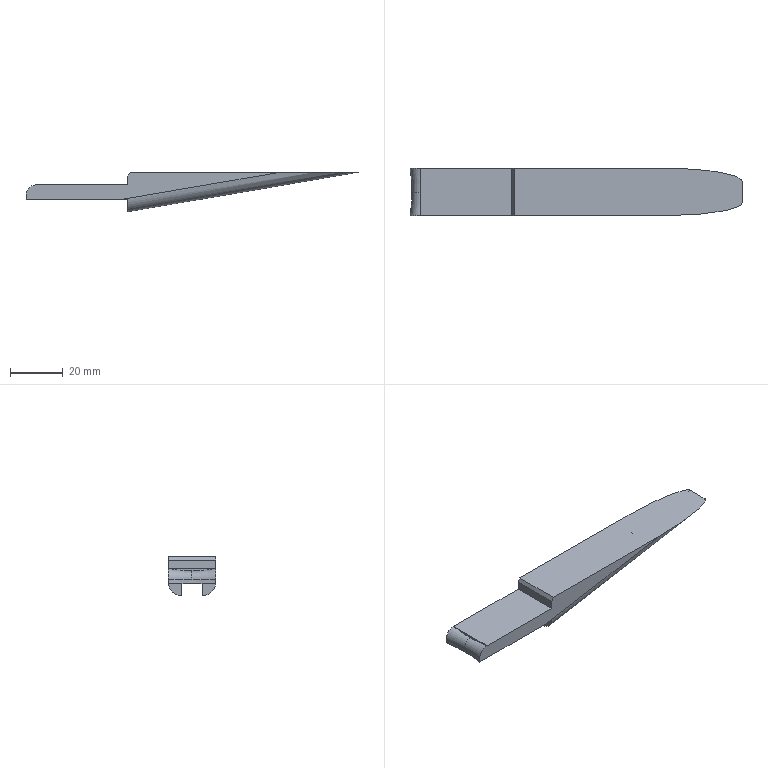Component | SolidWorks | Pata1-11-SW-1 | 1 solid | 28 faces | box 126.2 x 18 x 15 mm | volume 12034 mm3 | plane 21 | cylinder 5 | torus 2 | commonest cylinder face diameters 8 x2 10 x2 100 x1
STEP:
#1=COLOUR_RGB('',0.7922,0.8196,0.9333);
#2=FILL_AREA_STYLE_COLOUR('',#1);
#3=FILL_AREA_STYLE('',(#2));
#4=SURFACE_STYLE_FILL_AREA(#3);
#5=SURFACE_SIDE_STYLE('',(#4));
#6=SURFACE_STYLE_USAGE(.BOTH.,#5);
#7=PRESENTATION_STYLE_ASSIGNMENT((#6));
#8=CARTESIAN_POINT('',(-1.782,-0.7446,41.425));
#9=VERTEX_POINT('',#8);
#10=CARTESIAN_POINT('',(-1.782,-1.099,41.457));
#11=VERTEX_POINT('',#10);
#12=CARTESIAN_POINT('',(-1.782,-0.7446,43.393));
#13=DIRECTION('',(-1.,0.,0.));
#14=DIRECTION('',(-0.,-1.,0.));
#15=AXIS2_PLACEMENT_3D('',#12,#13,#14);
#16=CIRCLE('',#15,1.969);
#17=EDGE_CURVE('',#9,#11,#16,.T.);
#18=ORIENTED_EDGE('',*,*,#17,.F.);
#19=CARTESIAN_POINT('',(-1.908,-0.7446,41.299));
#20=VERTEX_POINT('',#19);
#21=CARTESIAN_POINT('',(-1.782,-0.7446,41.299));
#22=DIRECTION('',(-0.,-1.,-0.));
#23=DIRECTION('',(0.,0.,-1.));
#24=AXIS2_PLACEMENT_3D('',#21,#22,#23);
#25=CIRCLE('',#24,0.1253);
#26=EDGE_CURVE('',#9,#20,#25,.T.);
#27=ORIENTED_EDGE('',*,*,#26,.T.);
#28=CARTESIAN_POINT('',(-1.94,-1.099,41.299));
#29=VERTEX_POINT('',#28);
#30=CARTESIAN_POINT('',(-3.876,-0.7446,41.299));
#31=DIRECTION('',(-0.,0.,-1.));
#32=DIRECTION('',(0.,-1.,0.));
#33=AXIS2_PLACEMENT_3D('',#30,#31,#32);
#34=CIRCLE('',#33,1.969);
#35=EDGE_CURVE('',#20,#29,#34,.T.);
#36=ORIENTED_EDGE('',*,*,#35,.T.);
#37=CARTESIAN_POINT('',(-1.782,-1.099,41.299));
#38=DIRECTION('',(-0.,-1.,-0.));
#39=DIRECTION('',(1.,0.,0.));
#40=AXIS2_PLACEMENT_3D('',#37,#38,#39);
#41=CIRCLE('',#40,0.1575);
#42=EDGE_CURVE('',#11,#29,#41,.T.);
#43=ORIENTED_EDGE('',*,*,#42,.F.);
#44=EDGE_LOOP('',(#18,#27,#36,#43));
#45=FACE_OUTER_BOUND('',#44,.T.);
#46=CARTESIAN_POINT('',(-1.782,-0.7446,41.299));
#47=DIRECTION('',(-0.,-1.,-0.));
#48=DIRECTION('',(-1.,0.,-0.));
#49=AXIS2_PLACEMENT_3D('',#46,#47,#48);
#50=TOROIDAL_SURFACE('',#49,2.094,1.969);
#51=ADVANCED_FACE('',(#45),#50,.F.);
#52=CARTESIAN_POINT('',(-1.94,-0.3902,41.234));
#53=VERTEX_POINT('',#52);
#54=CARTESIAN_POINT('',(-1.94,-1.099,41.234));
#55=VERTEX_POINT('',#54);
#56=CARTESIAN_POINT('',(-3.876,-0.7446,41.234));
#57=DIRECTION('',(-0.,0.,-1.));
#58=DIRECTION('',(0.,1.,0.));
#59=AXIS2_PLACEMENT_3D('',#56,#57,#58);
#60=CIRCLE('',#59,1.969);
#61=EDGE_CURVE('',#53,#55,#60,.T.);
#62=ORIENTED_EDGE('',*,*,#61,.F.);
#63=CARTESIAN_POINT('',(-0.5249,-0.3902,41.234));
#64=VERTEX_POINT('',#63);
#65=CARTESIAN_POINT('',(-0.4163,-0.3902,41.234));
#66=DIRECTION('',(1.,-0.,-0.));
#67=VECTOR('',#66,39.37);
#68=LINE('',#65,#67);
#69=EDGE_CURVE('',#53,#64,#68,.T.);
#70=ORIENTED_EDGE('',*,*,#69,.T.);
#71=CARTESIAN_POINT('',(-0.4163,-0.3911,41.234));
#72=VERTEX_POINT('',#71);
#73=CARTESIAN_POINT('',(-0.5249,-0.3902,41.234));
#74=CARTESIAN_POINT('',(-0.4887,-0.3902,41.234));
#75=CARTESIAN_POINT('',(-0.4524,-0.3905,41.234));
#76=CARTESIAN_POINT('',(-0.4163,-0.3911,41.234));
#77=(BOUNDED_CURVE()B_SPLINE_CURVE(3,(#73,#74,#75,#76),.UNSPECIFIED.,.F.,.F.)B_SPLINE_CURVE_WITH_KNOTS((4,4),(1.571,1.664),.UNSPECIFIED.)CURVE()GEOMETRIC_REPRESENTATION_ITEM()RATIONAL_B_SPLINE_CURVE((1.,0.9993,0.9993,1.))REPRESENTATION_ITEM(''));
#78=EDGE_CURVE('',#64,#72,#77,.T.);
#79=ORIENTED_EDGE('',*,*,#78,.T.);
#80=CARTESIAN_POINT('',(-0.4163,-0.5914,41.234));
#81=VERTEX_POINT('',#80);
#82=CARTESIAN_POINT('',(-0.4163,-1.099,41.234));
#83=DIRECTION('',(0.,1.,0.));
#84=VECTOR('',#83,39.37);
#85=LINE('',#82,#84);
#86=EDGE_CURVE('',#81,#72,#85,.T.);
#87=ORIENTED_EDGE('',*,*,#86,.F.);
#88=CARTESIAN_POINT('',(-0.4163,-0.8978,41.234));
#89=VERTEX_POINT('',#88);
#90=CARTESIAN_POINT('',(-0.4163,-0.8978,41.234));
#91=CARTESIAN_POINT('',(-1.936,-0.8493,41.234));
#92=CARTESIAN_POINT('',(-1.936,-0.6399,41.234));
#93=CARTESIAN_POINT('',(-0.4163,-0.5914,41.234));
#94=(BOUNDED_CURVE()B_SPLINE_CURVE(3,(#90,#91,#92,#93),.UNSPECIFIED.,.F.,.F.)B_SPLINE_CURVE_WITH_KNOTS((4,4),(4.946,7.62),.UNSPECIFIED.)CURVE()GEOMETRIC_REPRESENTATION_ITEM()RATIONAL_B_SPLINE_CURVE((1.,0.4877,0.4877,1.))REPRESENTATION_ITEM(''));
#95=EDGE_CURVE('',#89,#81,#94,.T.);
#96=ORIENTED_EDGE('',*,*,#95,.F.);
#97=CARTESIAN_POINT('',(-0.4163,-1.098,41.234));
#98=VERTEX_POINT('',#97);
#99=CARTESIAN_POINT('',(-0.4163,-1.099,41.234));
#100=DIRECTION('',(0.,1.,0.));
#101=VECTOR('',#100,39.37);
#102=LINE('',#99,#101);
#103=EDGE_CURVE('',#98,#89,#102,.T.);
#104=ORIENTED_EDGE('',*,*,#103,.F.);
#105=CARTESIAN_POINT('',(-0.5249,-1.099,41.234));
#106=VERTEX_POINT('',#105);
#107=CARTESIAN_POINT('',(-0.4163,-1.098,41.234));
#108=CARTESIAN_POINT('',(-0.4524,-1.099,41.234));
#109=CARTESIAN_POINT('',(-0.4887,-1.099,41.234));
#110=CARTESIAN_POINT('',(-0.5249,-1.099,41.234));
#111=(BOUNDED_CURVE()B_SPLINE_CURVE(3,(#107,#108,#109,#110),.UNSPECIFIED.,.F.,.T.)B_SPLINE_CURVE_WITH_KNOTS((4,4),(1.477,1.571),.UNSPECIFIED.)CURVE()GEOMETRIC_REPRESENTATION_ITEM()RATIONAL_B_SPLINE_CURVE((1.,0.9993,0.9993,1.))REPRESENTATION_ITEM(''));
#112=EDGE_CURVE('',#98,#106,#111,.T.);
#113=ORIENTED_EDGE('',*,*,#112,.T.);
#114=CARTESIAN_POINT('',(-0.4163,-1.099,41.234));
#115=DIRECTION('',(1.,-0.,-0.));
#116=VECTOR('',#115,39.37);
#117=LINE('',#114,#116);
#118=EDGE_CURVE('',#55,#106,#117,.T.);
#119=ORIENTED_EDGE('',*,*,#118,.F.);
#120=EDGE_LOOP('',(#62,#70,#79,#87,#96,#104,#113,#119));
#121=FACE_OUTER_BOUND('',#120,.T.);
#122=CARTESIAN_POINT('',(-0.4163,-1.099,41.234));
#123=DIRECTION('',(0.,-0.,1.));
#124=DIRECTION('',(0.,1.,0.));
#125=AXIS2_PLACEMENT_3D('',#122,#123,#124);
#126=PLANE('',#125);
#127=ADVANCED_FACE('',(#121),#126,.F.);
#128=CARTESIAN_POINT('',(1.655,-0.5872,41.483));
#129=VERTEX_POINT('',#128);
#130=CARTESIAN_POINT('',(1.655,-0.5871,41.478));
#131=VERTEX_POINT('',#130);
#132=CARTESIAN_POINT('',(1.655,-0.5872,41.483));
#133=CARTESIAN_POINT('',(1.655,-0.5871,41.481));
#134=CARTESIAN_POINT('',(1.655,-0.5871,41.479));
#135=CARTESIAN_POINT('',(1.655,-0.5871,41.478));
#136=(BOUNDED_CURVE()B_SPLINE_CURVE(3,(#132,#133,#134,#135),.UNSPECIFIED.,.F.,.F.)B_SPLINE_CURVE_WITH_KNOTS((4,4),(4.679,4.712),.UNSPECIFIED.)CURVE()GEOMETRIC_REPRESENTATION_ITEM()RATIONAL_B_SPLINE_CURVE((1.,0.9999,0.9999,1.))REPRESENTATION_ITEM(''));
#137=EDGE_CURVE('',#129,#131,#136,.T.);
#138=ORIENTED_EDGE('',*,*,#137,.F.);
#139=CARTESIAN_POINT('',(1.655,-0.5871,41.483));
#140=VERTEX_POINT('',#139);
#141=CARTESIAN_POINT('',(1.655,-0.5871,41.483));
#142=DIRECTION('',(-0.,-1.,-0.));
#143=VECTOR('',#142,39.37);
#144=LINE('',#141,#143);
#145=EDGE_CURVE('',#140,#129,#144,.T.);
#146=ORIENTED_EDGE('',*,*,#145,.F.);
#147=CARTESIAN_POINT('',(1.655,-0.5871,41.408));
#148=DIRECTION('',(0.,-0.,1.));
#149=VECTOR('',#148,39.37);
#150=LINE('',#147,#149);
#151=EDGE_CURVE('',#131,#140,#150,.T.);
#152=ORIENTED_EDGE('',*,*,#151,.F.);
#153=EDGE_LOOP('',(#138,#146,#152));
#154=FACE_OUTER_BOUND('',#153,.T.);
#155=CARTESIAN_POINT('',(1.655,-0.5871,41.408));
#156=DIRECTION('',(1.,-0.,-0.));
#157=DIRECTION('',(-0.,-1.,-0.));
#158=AXIS2_PLACEMENT_3D('',#155,#156,#157);
#159=PLANE('',#158);
#160=ADVANCED_FACE('',(#154),#159,.F.);
#161=CARTESIAN_POINT('',(1.655,-0.9018,41.469));
#162=VERTEX_POINT('',#161);
#163=CARTESIAN_POINT('',(1.655,-0.902,41.478));
#164=VERTEX_POINT('',#163);
#165=CARTESIAN_POINT('',(1.655,-0.9018,41.469));
#166=CARTESIAN_POINT('',(1.655,-0.902,41.472));
#167=CARTESIAN_POINT('',(1.655,-0.902,41.475));
#168=CARTESIAN_POINT('',(1.655,-0.902,41.478));
#169=(BOUNDED_CURVE()B_SPLINE_CURVE(3,(#165,#166,#167,#168),.UNSPECIFIED.,.F.,.T.)B_SPLINE_CURVE_WITH_KNOTS((4,4),(1.519,1.571),.UNSPECIFIED.)CURVE()GEOMETRIC_REPRESENTATION_ITEM()RATIONAL_B_SPLINE_CURVE((1.,0.9998,0.9998,1.))REPRESENTATION_ITEM(''));
#170=EDGE_CURVE('',#162,#164,#169,.T.);
#171=ORIENTED_EDGE('',*,*,#170,.F.);
#172=CARTESIAN_POINT('',(1.655,-0.902,41.408));
#173=VERTEX_POINT('',#172);
#174=CARTESIAN_POINT('',(1.655,-0.902,41.408));
#175=CARTESIAN_POINT('',(1.655,-0.902,41.429));
#176=CARTESIAN_POINT('',(1.655,-0.902,41.449));
#177=CARTESIAN_POINT('',(1.655,-0.9018,41.469));
#178=(BOUNDED_CURVE()B_SPLINE_CURVE(3,(#174,#175,#176,#177),.UNSPECIFIED.,.F.,.F.)B_SPLINE_CURVE_WITH_KNOTS((4,4),(4.712,4.765),.UNSPECIFIED.)CURVE()GEOMETRIC_REPRESENTATION_ITEM()RATIONAL_B_SPLINE_CURVE((1.,0.9998,0.9998,1.))REPRESENTATION_ITEM(''));
#179=EDGE_CURVE('',#173,#162,#178,.T.);
#180=ORIENTED_EDGE('',*,*,#179,.F.);
#181=CARTESIAN_POINT('',(1.655,-0.902,41.408));
#182=DIRECTION('',(0.,-0.,1.));
#183=VECTOR('',#182,39.37);
#184=LINE('',#181,#183);
#185=EDGE_CURVE('',#173,#164,#184,.T.);
#186=ORIENTED_EDGE('',*,*,#185,.T.);
#187=EDGE_LOOP('',(#171,#180,#186));
#188=FACE_OUTER_BOUND('',#187,.T.);
#189=CARTESIAN_POINT('',(1.655,-0.5871,41.408));
#190=DIRECTION('',(1.,-0.,-0.));
#191=DIRECTION('',(-0.,-1.,-0.));
#192=AXIS2_PLACEMENT_3D('',#189,#190,#191);
#193=PLANE('',#192);
#194=ADVANCED_FACE('',(#188),#193,.F.);
#195=CARTESIAN_POINT('',(-0.4163,-0.902,41.203));
#196=VERTEX_POINT('',#195);
#197=CARTESIAN_POINT('',(-0.4163,-0.902,41.203));
#198=CARTESIAN_POINT('',(-0.4163,-0.9016,41.213));
#199=CARTESIAN_POINT('',(-0.4163,-0.9002,41.224));
#200=CARTESIAN_POINT('',(-0.4163,-0.8978,41.234));
#201=(BOUNDED_CURVE()B_SPLINE_CURVE(3,(#197,#198,#199,#200),.UNSPECIFIED.,.F.,.F.)B_SPLINE_CURVE_WITH_KNOTS((4,4),(1.604,1.805),.UNSPECIFIED.)CURVE()GEOMETRIC_REPRESENTATION_ITEM()RATIONAL_B_SPLINE_CURVE((1.,0.9967,0.9967,1.))REPRESENTATION_ITEM(''));
#202=EDGE_CURVE('',#196,#89,#201,.T.);
#203=ORIENTED_EDGE('',*,*,#202,.F.);
#204=CARTESIAN_POINT('',(-0.4163,-0.902,41.203));
#205=VERTEX_POINT('',#204);
#206=CARTESIAN_POINT('',(-0.4163,-0.5871,41.203));
#207=DIRECTION('',(-0.,-1.,-0.));
#208=VECTOR('',#207,39.37);
#209=LINE('',#206,#208);
#210=EDGE_CURVE('',#196,#205,#209,.T.);
#211=ORIENTED_EDGE('',*,*,#210,.T.);
#212=CARTESIAN_POINT('',(-0.4163,-0.902,41.053));
#213=VERTEX_POINT('',#212);
#214=CARTESIAN_POINT('',(-0.4163,-0.902,41.234));
#215=DIRECTION('',(-0.,0.,-1.));
#216=VECTOR('',#215,39.37);
#217=LINE('',#214,#216);
#218=EDGE_CURVE('',#205,#213,#217,.T.);
#219=ORIENTED_EDGE('',*,*,#218,.T.);
#220=CARTESIAN_POINT('',(-0.4163,-0.902,41.053));
#221=CARTESIAN_POINT('',(-0.4163,-1.009,41.053));
#222=CARTESIAN_POINT('',(-0.4163,-1.088,41.126));
#223=CARTESIAN_POINT('',(-0.4163,-1.098,41.234));
#224=(BOUNDED_CURVE()B_SPLINE_CURVE(3,(#220,#221,#222,#223),.UNSPECIFIED.,.F.,.F.)B_SPLINE_CURVE_WITH_KNOTS((4,4),(3.142,4.619),.UNSPECIFIED.)CURVE()GEOMETRIC_REPRESENTATION_ITEM()RATIONAL_B_SPLINE_CURVE((1.,0.8262,0.8262,1.))REPRESENTATION_ITEM(''));
#225=EDGE_CURVE('',#213,#98,#224,.T.);
#226=ORIENTED_EDGE('',*,*,#225,.T.);
#227=ORIENTED_EDGE('',*,*,#103,.T.);
#228=EDGE_LOOP('',(#203,#211,#219,#226,#227));
#229=FACE_OUTER_BOUND('',#228,.T.);
#230=CARTESIAN_POINT('',(-0.4163,-1.099,41.234));
#231=DIRECTION('',(1.,-0.,-0.));
#232=DIRECTION('',(-0.,-1.,-0.));
#233=AXIS2_PLACEMENT_3D('',#230,#231,#232);
#234=PLANE('',#233);
#235=ADVANCED_FACE('',(#229),#234,.F.);
#236=CARTESIAN_POINT('',(-0.4163,-0.5872,41.203));
#237=VERTEX_POINT('',#236);
#238=CARTESIAN_POINT('',(1.655,-0.5872,41.483));
#239=DIRECTION('',(0.991,-0.,0.1341));
#240=VECTOR('',#239,39.37);
#241=LINE('',#238,#240);
#242=EDGE_CURVE('',#237,#129,#241,.T.);
#243=ORIENTED_EDGE('',*,*,#242,.F.);
#244=CARTESIAN_POINT('',(-0.4163,-0.5871,41.203));
#245=VERTEX_POINT('',#244);
#246=CARTESIAN_POINT('',(-0.4163,-0.5871,41.203));
#247=DIRECTION('',(-0.,-1.,-0.));
#248=VECTOR('',#247,39.37);
#249=LINE('',#246,#248);
#250=EDGE_CURVE('',#245,#237,#249,.T.);
#251=ORIENTED_EDGE('',*,*,#250,.F.);
#252=CARTESIAN_POINT('',(1.655,-0.5871,41.483));
#253=DIRECTION('',(-0.991,0.,-0.1341));
#254=VECTOR('',#253,39.37);
#255=LINE('',#252,#254);
#256=EDGE_CURVE('',#140,#245,#255,.T.);
#257=ORIENTED_EDGE('',*,*,#256,.F.);
#258=ORIENTED_EDGE('',*,*,#145,.T.);
#259=EDGE_LOOP('',(#243,#251,#257,#258));
#260=FACE_OUTER_BOUND('',#259,.T.);
#261=CARTESIAN_POINT('',(1.655,-0.5871,41.483));
#262=DIRECTION('',(-0.1341,-0.,0.991));
#263=DIRECTION('',(-0.991,0.,-0.1341));
#264=AXIS2_PLACEMENT_3D('',#261,#262,#263);
#265=PLANE('',#264);
#266=ADVANCED_FACE('',(#260),#265,.F.);
#267=CARTESIAN_POINT('',(1.655,-0.902,41.483));
#268=VERTEX_POINT('',#267);
#269=CARTESIAN_POINT('',(1.655,-0.902,41.483));
#270=DIRECTION('',(-0.991,0.,-0.1341));
#271=VECTOR('',#270,39.37);
#272=LINE('',#269,#271);
#273=EDGE_CURVE('',#268,#196,#272,.T.);
#274=ORIENTED_EDGE('',*,*,#273,.F.);
#275=CARTESIAN_POINT('',(1.655,-0.902,41.483));
#276=VERTEX_POINT('',#275);
#277=CARTESIAN_POINT('',(1.655,-0.5871,41.483));
#278=DIRECTION('',(-0.,-1.,-0.));
#279=VECTOR('',#278,39.37);
#280=LINE('',#277,#279);
#281=EDGE_CURVE('',#268,#276,#280,.T.);
#282=ORIENTED_EDGE('',*,*,#281,.T.);
#283=CARTESIAN_POINT('',(1.655,-0.902,41.483));
#284=DIRECTION('',(-0.991,0.,-0.1341));
#285=VECTOR('',#284,39.37);
#286=LINE('',#283,#285);
#287=EDGE_CURVE('',#276,#205,#286,.T.);
#288=ORIENTED_EDGE('',*,*,#287,.T.);
#289=ORIENTED_EDGE('',*,*,#210,.F.);
#290=EDGE_LOOP('',(#274,#282,#288,#289));
#291=FACE_OUTER_BOUND('',#290,.T.);
#292=CARTESIAN_POINT('',(1.655,-0.5871,41.483));
#293=DIRECTION('',(-0.1341,-0.,0.991));
#294=DIRECTION('',(-0.991,0.,-0.1341));
#295=AXIS2_PLACEMENT_3D('',#292,#293,#294);
#296=PLANE('',#295);
#297=ADVANCED_FACE('',(#291),#296,.F.);
#298=CARTESIAN_POINT('',(1.658,-0.5875,41.467));
#299=VERTEX_POINT('',#298);
#300=CARTESIAN_POINT('',(1.655,-0.5875,41.483));
#301=VERTEX_POINT('',#300);
#302=CARTESIAN_POINT('',(1.666,-0.5875,41.405));
#303=DIRECTION('',(-0.1341,-0.,0.991));
#304=VECTOR('',#303,39.37);
#305=LINE('',#302,#304);
#306=EDGE_CURVE('',#299,#301,#305,.T.);
#307=ORIENTED_EDGE('',*,*,#306,.F.);
#308=CARTESIAN_POINT('',(1.655,-0.5873,41.469));
#309=VERTEX_POINT('',#308);
#310=CARTESIAN_POINT('',(1.658,-0.5875,41.467));
#311=CARTESIAN_POINT('',(1.657,-0.5874,41.468));
#312=CARTESIAN_POINT('',(1.656,-0.5873,41.469));
#313=CARTESIAN_POINT('',(1.655,-0.5873,41.469));
#314=(BOUNDED_CURVE()B_SPLINE_CURVE(3,(#310,#311,#312,#313),.UNSPECIFIED.,.F.,.F.)B_SPLINE_CURVE_WITH_KNOTS((4,4),(4.643,4.66),.UNSPECIFIED.)CURVE()GEOMETRIC_REPRESENTATION_ITEM()RATIONAL_B_SPLINE_CURVE((1.,1.,1.,1.))REPRESENTATION_ITEM(''));
#315=EDGE_CURVE('',#299,#309,#314,.T.);
#316=ORIENTED_EDGE('',*,*,#315,.T.);
#317=CARTESIAN_POINT('',(1.655,-0.5871,41.408));
#318=VERTEX_POINT('',#317);
#319=CARTESIAN_POINT('',(1.655,-0.5873,41.469));
#320=CARTESIAN_POINT('',(1.655,-0.5871,41.449));
#321=CARTESIAN_POINT('',(1.655,-0.5871,41.429));
#322=CARTESIAN_POINT('',(1.655,-0.5871,41.408));
#323=(BOUNDED_CURVE()B_SPLINE_CURVE(3,(#319,#320,#321,#322),.UNSPECIFIED.,.F.,.F.)B_SPLINE_CURVE_WITH_KNOTS((4,4),(1.519,1.571),.UNSPECIFIED.)CURVE()GEOMETRIC_REPRESENTATION_ITEM()RATIONAL_B_SPLINE_CURVE((1.,0.9998,0.9998,1.))REPRESENTATION_ITEM(''));
#324=EDGE_CURVE('',#309,#318,#323,.T.);
#325=ORIENTED_EDGE('',*,*,#324,.T.);
#326=CARTESIAN_POINT('',(1.655,-0.5871,41.408));
#327=CARTESIAN_POINT('',(1.965,-0.5871,41.461));
#328=CARTESIAN_POINT('',(1.965,-0.902,41.461));
#329=CARTESIAN_POINT('',(1.655,-0.902,41.408));
#330=(BOUNDED_CURVE()B_SPLINE_CURVE(3,(#326,#327,#328,#329),.UNSPECIFIED.,.F.,.F.)B_SPLINE_CURVE_WITH_KNOTS((4,4),(4.712,7.854),.UNSPECIFIED.)CURVE()GEOMETRIC_REPRESENTATION_ITEM()RATIONAL_B_SPLINE_CURVE((1.,0.3333,0.3333,1.))REPRESENTATION_ITEM(''));
#331=EDGE_CURVE('',#318,#173,#330,.T.);
#332=ORIENTED_EDGE('',*,*,#331,.T.);
#333=ORIENTED_EDGE('',*,*,#179,.T.);
#334=CARTESIAN_POINT('',(1.658,-0.9017,41.467));
#335=VERTEX_POINT('',#334);
#336=CARTESIAN_POINT('',(1.655,-0.9018,41.469));
#337=CARTESIAN_POINT('',(1.656,-0.9018,41.469));
#338=CARTESIAN_POINT('',(1.657,-0.9017,41.468));
#339=CARTESIAN_POINT('',(1.658,-0.9017,41.467));
#340=(BOUNDED_CURVE()B_SPLINE_CURVE(3,(#336,#337,#338,#339),.UNSPECIFIED.,.F.,.F.)B_SPLINE_CURVE_WITH_KNOTS((4,4),(1.623,1.64),.UNSPECIFIED.)CURVE()GEOMETRIC_REPRESENTATION_ITEM()RATIONAL_B_SPLINE_CURVE((1.,1.,1.,1.))REPRESENTATION_ITEM(''));
#341=EDGE_CURVE('',#162,#335,#340,.T.);
#342=ORIENTED_EDGE('',*,*,#341,.T.);
#343=CARTESIAN_POINT('',(1.655,-0.9017,41.483));
#344=VERTEX_POINT('',#343);
#345=CARTESIAN_POINT('',(1.666,-0.9017,41.405));
#346=DIRECTION('',(0.1341,0.,-0.991));
#347=VECTOR('',#346,39.37);
#348=LINE('',#345,#347);
#349=EDGE_CURVE('',#344,#335,#348,.T.);
#350=ORIENTED_EDGE('',*,*,#349,.F.);
#351=CARTESIAN_POINT('',(1.645,-0.7446,41.482));
#352=DIRECTION('',(0.1341,0.,-0.991));
#353=DIRECTION('',(0.991,0.,0.1341));
#354=AXIS2_PLACEMENT_3D('',#351,#352,#353);
#355=CIRCLE('',#354,0.1575);
#356=EDGE_CURVE('',#301,#344,#355,.T.);
#357=ORIENTED_EDGE('',*,*,#356,.F.);
#358=EDGE_LOOP('',(#307,#316,#325,#332,#333,#342,#350,#357));
#359=FACE_OUTER_BOUND('',#358,.T.);
#360=CARTESIAN_POINT('',(1.655,-0.7446,41.404));
#361=DIRECTION('',(-0.1341,-0.,0.991));
#362=DIRECTION('',(-0.991,0.,-0.1341));
#363=AXIS2_PLACEMENT_3D('',#360,#361,#362);
#364=CYLINDRICAL_SURFACE('',#363,0.1575);
#365=ADVANCED_FACE('',(#359),#364,.F.);
#366=CARTESIAN_POINT('',(1.655,-0.5871,41.478));
#367=CARTESIAN_POINT('',(1.655,-0.5871,41.475));
#368=CARTESIAN_POINT('',(1.655,-0.5871,41.472));
#369=CARTESIAN_POINT('',(1.655,-0.5873,41.469));
#370=(BOUNDED_CURVE()B_SPLINE_CURVE(3,(#366,#367,#368,#369),.UNSPECIFIED.,.F.,.F.)B_SPLINE_CURVE_WITH_KNOTS((4,4),(4.712,4.765),.UNSPECIFIED.)CURVE()GEOMETRIC_REPRESENTATION_ITEM()RATIONAL_B_SPLINE_CURVE((1.,0.9998,0.9998,1.))REPRESENTATION_ITEM(''));
#371=EDGE_CURVE('',#131,#309,#370,.T.);
#372=ORIENTED_EDGE('',*,*,#371,.F.);
#373=CARTESIAN_POINT('',(1.655,-0.5871,41.408));
#374=DIRECTION('',(0.,-0.,1.));
#375=VECTOR('',#374,39.37);
#376=LINE('',#373,#375);
#377=EDGE_CURVE('',#318,#131,#376,.T.);
#378=ORIENTED_EDGE('',*,*,#377,.F.);
#379=ORIENTED_EDGE('',*,*,#324,.F.);
#380=EDGE_LOOP('',(#372,#378,#379));
#381=FACE_OUTER_BOUND('',#380,.T.);
#382=CARTESIAN_POINT('',(1.655,-0.5871,41.408));
#383=DIRECTION('',(1.,-0.,-0.));
#384=DIRECTION('',(-0.,-1.,-0.));
#385=AXIS2_PLACEMENT_3D('',#382,#383,#384);
#386=PLANE('',#385);
#387=ADVANCED_FACE('',(#381),#386,.F.);
#388=CARTESIAN_POINT('',(1.655,-0.902,41.478));
#389=CARTESIAN_POINT('',(1.655,-0.902,41.479));
#390=CARTESIAN_POINT('',(1.655,-0.902,41.481));
#391=CARTESIAN_POINT('',(1.655,-0.902,41.483));
#392=(BOUNDED_CURVE()B_SPLINE_CURVE(3,(#388,#389,#390,#391),.UNSPECIFIED.,.F.,.F.)B_SPLINE_CURVE_WITH_KNOTS((4,4),(1.571,1.604),.UNSPECIFIED.)CURVE()GEOMETRIC_REPRESENTATION_ITEM()RATIONAL_B_SPLINE_CURVE((1.,0.9999,0.9999,1.))REPRESENTATION_ITEM(''));
#393=EDGE_CURVE('',#164,#268,#392,.T.);
#394=ORIENTED_EDGE('',*,*,#393,.F.);
#395=CARTESIAN_POINT('',(1.655,-0.902,41.408));
#396=DIRECTION('',(0.,-0.,1.));
#397=VECTOR('',#396,39.37);
#398=LINE('',#395,#397);
#399=EDGE_CURVE('',#164,#276,#398,.T.);
#400=ORIENTED_EDGE('',*,*,#399,.T.);
#401=ORIENTED_EDGE('',*,*,#281,.F.);
#402=EDGE_LOOP('',(#394,#400,#401));
#403=FACE_OUTER_BOUND('',#402,.T.);
#404=CARTESIAN_POINT('',(1.655,-0.5871,41.408));
#405=DIRECTION('',(1.,-0.,-0.));
#406=DIRECTION('',(-0.,-1.,-0.));
#407=AXIS2_PLACEMENT_3D('',#404,#405,#406);
#408=PLANE('',#407);
#409=ADVANCED_FACE('',(#403),#408,.F.);
#410=ORIENTED_EDGE('',*,*,#331,.F.);
#411=CARTESIAN_POINT('',(3.029,-0.5871,41.644));
#412=VERTEX_POINT('',#411);
#413=CARTESIAN_POINT('',(3.029,-0.5871,41.644));
#414=DIRECTION('',(0.9856,-0.,0.169));
#415=VECTOR('',#414,39.37);
#416=LINE('',#413,#415);
#417=EDGE_CURVE('',#318,#412,#416,.T.);
#418=ORIENTED_EDGE('',*,*,#417,.T.);
#419=CARTESIAN_POINT('',(3.029,-0.902,41.644));
#420=VERTEX_POINT('',#419);
#421=CARTESIAN_POINT('',(3.029,-1.099,41.644));
#422=DIRECTION('',(0.,1.,0.));
#423=VECTOR('',#422,39.37);
#424=LINE('',#421,#423);
#425=EDGE_CURVE('',#420,#412,#424,.T.);
#426=ORIENTED_EDGE('',*,*,#425,.F.);
#427=CARTESIAN_POINT('',(-0.4163,-0.902,41.053));
#428=DIRECTION('',(-0.9856,0.,-0.169));
#429=VECTOR('',#428,39.37);
#430=LINE('',#427,#429);
#431=EDGE_CURVE('',#420,#173,#430,.T.);
#432=ORIENTED_EDGE('',*,*,#431,.T.);
#433=EDGE_LOOP('',(#410,#418,#426,#432));
#434=FACE_OUTER_BOUND('',#433,.T.);
#435=CARTESIAN_POINT('',(-0.4163,-1.099,41.053));
#436=DIRECTION('',(-0.169,-0.,0.9856));
#437=DIRECTION('',(-0.9856,0.,-0.169));
#438=AXIS2_PLACEMENT_3D('',#435,#436,#437);
#439=PLANE('',#438);
#440=ADVANCED_FACE('',(#434),#439,.F.);
#441=CARTESIAN_POINT('',(-0.4163,-0.5914,41.234));
#442=CARTESIAN_POINT('',(-0.4163,-0.5889,41.224));
#443=CARTESIAN_POINT('',(-0.4163,-0.5875,41.213));
#444=CARTESIAN_POINT('',(-0.4163,-0.5872,41.203));
#445=(BOUNDED_CURVE()B_SPLINE_CURVE(3,(#441,#442,#443,#444),.UNSPECIFIED.,.F.,.F.)B_SPLINE_CURVE_WITH_KNOTS((4,4),(4.479,4.679),.UNSPECIFIED.)CURVE()GEOMETRIC_REPRESENTATION_ITEM()RATIONAL_B_SPLINE_CURVE((1.,0.9967,0.9967,1.))REPRESENTATION_ITEM(''));
#446=EDGE_CURVE('',#81,#237,#445,.T.);
#447=ORIENTED_EDGE('',*,*,#446,.F.);
#448=ORIENTED_EDGE('',*,*,#86,.T.);
#449=CARTESIAN_POINT('',(-0.4163,-0.5871,41.053));
#450=VERTEX_POINT('',#449);
#451=CARTESIAN_POINT('',(-0.4163,-0.3911,41.234));
#452=CARTESIAN_POINT('',(-0.4163,-0.4011,41.126));
#453=CARTESIAN_POINT('',(-0.4163,-0.4801,41.053));
#454=CARTESIAN_POINT('',(-0.4163,-0.5871,41.053));
#455=(BOUNDED_CURVE()B_SPLINE_CURVE(3,(#451,#452,#453,#454),.UNSPECIFIED.,.F.,.F.)B_SPLINE_CURVE_WITH_KNOTS((4,4),(4.806,6.283),.UNSPECIFIED.)CURVE()GEOMETRIC_REPRESENTATION_ITEM()RATIONAL_B_SPLINE_CURVE((1.,0.8262,0.8262,1.))REPRESENTATION_ITEM(''));
#456=EDGE_CURVE('',#72,#450,#455,.T.);
#457=ORIENTED_EDGE('',*,*,#456,.T.);
#458=CARTESIAN_POINT('',(-0.4163,-0.5871,41.234));
#459=DIRECTION('',(0.,-0.,1.));
#460=VECTOR('',#459,39.37);
#461=LINE('',#458,#460);
#462=EDGE_CURVE('',#450,#245,#461,.T.);
#463=ORIENTED_EDGE('',*,*,#462,.T.);
#464=ORIENTED_EDGE('',*,*,#250,.T.);
#465=EDGE_LOOP('',(#447,#448,#457,#463,#464));
#466=FACE_OUTER_BOUND('',#465,.T.);
#467=CARTESIAN_POINT('',(-0.4163,-1.099,41.234));
#468=DIRECTION('',(1.,-0.,-0.));
#469=DIRECTION('',(-0.,-1.,-0.));
#470=AXIS2_PLACEMENT_3D('',#467,#468,#469);
#471=PLANE('',#470);
#472=ADVANCED_FACE('',(#466),#471,.F.);
#473=CARTESIAN_POINT('',(1.864,-0.3902,41.644));
#474=VERTEX_POINT('',#473);
#475=CARTESIAN_POINT('',(-0.3822,-0.3902,41.644));
#476=VERTEX_POINT('',#475);
#477=CARTESIAN_POINT('',(3.029,-0.3902,41.644));
#478=DIRECTION('',(-1.,0.,0.));
#479=VECTOR('',#478,39.37);
#480=LINE('',#477,#479);
#481=EDGE_CURVE('',#474,#476,#480,.T.);
#482=ORIENTED_EDGE('',*,*,#481,.T.);
#483=CARTESIAN_POINT('',(-0.3822,-1.099,41.644));
#484=VERTEX_POINT('',#483);
#485=CARTESIAN_POINT('',(-0.3822,-1.099,41.644));
#486=DIRECTION('',(-0.,-1.,-0.));
#487=VECTOR('',#486,39.37);
#488=LINE('',#485,#487);
#489=EDGE_CURVE('',#476,#484,#488,.T.);
#490=ORIENTED_EDGE('',*,*,#489,.T.);
#491=CARTESIAN_POINT('',(1.864,-1.099,41.644));
#492=VERTEX_POINT('',#491);
#493=CARTESIAN_POINT('',(3.029,-1.099,41.644));
#494=DIRECTION('',(-1.,0.,0.));
#495=VECTOR('',#494,39.37);
#496=LINE('',#493,#495);
#497=EDGE_CURVE('',#492,#484,#496,.T.);
#498=ORIENTED_EDGE('',*,*,#497,.F.);
#499=CARTESIAN_POINT('',(1.864,-1.099,41.644));
#500=CARTESIAN_POINT('',(2.546,-1.099,41.644));
#501=CARTESIAN_POINT('',(3.029,-1.017,41.644));
#502=CARTESIAN_POINT('',(3.029,-0.902,41.644));
#503=(BOUNDED_CURVE()B_SPLINE_CURVE(3,(#499,#500,#501,#502),.UNSPECIFIED.,.F.,.F.)B_SPLINE_CURVE_WITH_KNOTS((4,4),(4.712,6.283),.UNSPECIFIED.)CURVE()GEOMETRIC_REPRESENTATION_ITEM()RATIONAL_B_SPLINE_CURVE((1.,0.8047,0.8047,1.))REPRESENTATION_ITEM(''));
#504=EDGE_CURVE('',#492,#420,#503,.T.);
#505=ORIENTED_EDGE('',*,*,#504,.T.);
#506=ORIENTED_EDGE('',*,*,#425,.T.);
#507=CARTESIAN_POINT('',(3.029,-0.5871,41.644));
#508=CARTESIAN_POINT('',(3.029,-0.4718,41.644));
#509=CARTESIAN_POINT('',(2.546,-0.3902,41.644));
#510=CARTESIAN_POINT('',(1.864,-0.3902,41.644));
#511=(BOUNDED_CURVE()B_SPLINE_CURVE(3,(#507,#508,#509,#510),.UNSPECIFIED.,.F.,.F.)B_SPLINE_CURVE_WITH_KNOTS((4,4),(3.142,4.712),.UNSPECIFIED.)CURVE()GEOMETRIC_REPRESENTATION_ITEM()RATIONAL_B_SPLINE_CURVE((1.,0.8047,0.8047,1.))REPRESENTATION_ITEM(''));
#512=EDGE_CURVE('',#412,#474,#511,.T.);
#513=ORIENTED_EDGE('',*,*,#512,.T.);
#514=EDGE_LOOP('',(#482,#490,#498,#505,#506,#513));
#515=FACE_OUTER_BOUND('',#514,.T.);
#516=CARTESIAN_POINT('',(3.029,-1.099,41.644));
#517=DIRECTION('',(-0.,0.,-1.));
#518=DIRECTION('',(-0.,-1.,-0.));
#519=AXIS2_PLACEMENT_3D('',#516,#517,#518);
#520=PLANE('',#519);
#521=ADVANCED_FACE('',(#515),#520,.F.);
#522=CARTESIAN_POINT('',(-0.4163,-1.099,41.585));
#523=VERTEX_POINT('',#522);
#524=CARTESIAN_POINT('',(-0.4163,-1.099,41.457));
#525=VERTEX_POINT('',#524);
#526=CARTESIAN_POINT('',(-0.4163,-1.099,41.644));
#527=DIRECTION('',(-0.,0.,-1.));
#528=VECTOR('',#527,39.37);
#529=LINE('',#526,#528);
#530=EDGE_CURVE('',#523,#525,#529,.T.);
#531=ORIENTED_EDGE('',*,*,#530,.F.);
#532=CARTESIAN_POINT('',(-0.4163,-0.3902,41.585));
#533=VERTEX_POINT('',#532);
#534=CARTESIAN_POINT('',(-0.4163,-1.099,41.585));
#535=DIRECTION('',(0.,1.,0.));
#536=VECTOR('',#535,39.37);
#537=LINE('',#534,#536);
#538=EDGE_CURVE('',#523,#533,#537,.T.);
#539=ORIENTED_EDGE('',*,*,#538,.T.);
#540=CARTESIAN_POINT('',(-0.4163,-0.3902,41.457));
#541=VERTEX_POINT('',#540);
#542=CARTESIAN_POINT('',(-0.4163,-0.3902,41.644));
#543=DIRECTION('',(-0.,0.,-1.));
#544=VECTOR('',#543,39.37);
#545=LINE('',#542,#544);
#546=EDGE_CURVE('',#533,#541,#545,.T.);
#547=ORIENTED_EDGE('',*,*,#546,.T.);
#548=CARTESIAN_POINT('',(-0.4163,-1.099,41.457));
#549=DIRECTION('',(0.,1.,0.));
#550=VECTOR('',#549,39.37);
#551=LINE('',#548,#550);
#552=EDGE_CURVE('',#525,#541,#551,.T.);
#553=ORIENTED_EDGE('',*,*,#552,.F.);
#554=EDGE_LOOP('',(#531,#539,#547,#553));
#555=FACE_OUTER_BOUND('',#554,.T.);
#556=CARTESIAN_POINT('',(-0.4163,-1.099,41.644));
#557=DIRECTION('',(1.,-0.,-0.));
#558=DIRECTION('',(-0.,-1.,-0.));
#559=AXIS2_PLACEMENT_3D('',#556,#557,#558);
#560=PLANE('',#559);
#561=ADVANCED_FACE('',(#555),#560,.F.);
#562=CARTESIAN_POINT('',(-1.782,-0.3902,41.457));
#563=VERTEX_POINT('',#562);
#564=CARTESIAN_POINT('',(-1.94,-0.3902,41.457));
#565=DIRECTION('',(-1.,0.,0.));
#566=VECTOR('',#565,39.37);
#567=LINE('',#564,#566);
#568=EDGE_CURVE('',#541,#563,#567,.T.);
#569=ORIENTED_EDGE('',*,*,#568,.T.);
#570=CARTESIAN_POINT('',(-1.782,-1.099,41.457));
#571=DIRECTION('',(-0.,-1.,-0.));
#572=VECTOR('',#571,39.37);
#573=LINE('',#570,#572);
#574=EDGE_CURVE('',#563,#11,#573,.T.);
#575=ORIENTED_EDGE('',*,*,#574,.T.);
#576=CARTESIAN_POINT('',(-1.94,-1.099,41.457));
#577=DIRECTION('',(-1.,0.,0.));
#578=VECTOR('',#577,39.37);
#579=LINE('',#576,#578);
#580=EDGE_CURVE('',#525,#11,#579,.T.);
#581=ORIENTED_EDGE('',*,*,#580,.F.);
#582=ORIENTED_EDGE('',*,*,#552,.T.);
#583=EDGE_LOOP('',(#569,#575,#581,#582));
#584=FACE_OUTER_BOUND('',#583,.T.);
#585=CARTESIAN_POINT('',(-1.94,-1.099,41.457));
#586=DIRECTION('',(-0.,0.,-1.));
#587=DIRECTION('',(1.,-0.,-0.));
#588=AXIS2_PLACEMENT_3D('',#585,#586,#587);
#589=PLANE('',#588);
#590=ADVANCED_FACE('',(#584),#589,.F.);
#591=ORIENTED_EDGE('',*,*,#580,.T.);
#592=ORIENTED_EDGE('',*,*,#42,.T.);
#593=CARTESIAN_POINT('',(-1.94,-1.099,41.234));
#594=DIRECTION('',(-0.,0.,-1.));
#595=VECTOR('',#594,39.37);
#596=LINE('',#593,#595);
#597=EDGE_CURVE('',#29,#55,#596,.T.);
#598=ORIENTED_EDGE('',*,*,#597,.T.);
#599=ORIENTED_EDGE('',*,*,#118,.T.);
#600=CARTESIAN_POINT('',(2.995,-1.099,41.838));
#601=DIRECTION('',(0.9856,-0.,0.169));
#602=VECTOR('',#601,39.37);
#603=LINE('',#600,#602);
#604=EDGE_CURVE('',#106,#492,#603,.T.);
#605=ORIENTED_EDGE('',*,*,#604,.T.);
#606=ORIENTED_EDGE('',*,*,#497,.T.);
#607=CARTESIAN_POINT('',(-0.4163,-1.099,41.585));
#608=DIRECTION('',(-0.5,0.,-0.866));
#609=VECTOR('',#608,39.37);
#610=LINE('',#607,#609);
#611=EDGE_CURVE('',#484,#523,#610,.T.);
#612=ORIENTED_EDGE('',*,*,#611,.T.);
#613=ORIENTED_EDGE('',*,*,#530,.T.);
#614=EDGE_LOOP('',(#591,#592,#598,#599,#605,#606,#612,#613));
#615=FACE_OUTER_BOUND('',#614,.T.);
#616=CARTESIAN_POINT('',(3.029,-1.099,41.644));
#617=DIRECTION('',(0.,1.,0.));
#618=DIRECTION('',(1.,-0.,-0.));
#619=AXIS2_PLACEMENT_3D('',#616,#617,#618);
#620=PLANE('',#619);
#621=ADVANCED_FACE('',(#615),#620,.F.);
#622=CARTESIAN_POINT('',(-1.94,-0.3902,41.299));
#623=VERTEX_POINT('',#622);
#624=CARTESIAN_POINT('',(-1.94,-0.3902,41.234));
#625=DIRECTION('',(-0.,0.,-1.));
#626=VECTOR('',#625,39.37);
#627=LINE('',#624,#626);
#628=EDGE_CURVE('',#623,#53,#627,.T.);
#629=ORIENTED_EDGE('',*,*,#628,.F.);
#630=CARTESIAN_POINT('',(-1.782,-0.3902,41.299));
#631=DIRECTION('',(0.,1.,0.));
#632=DIRECTION('',(1.,0.,0.));
#633=AXIS2_PLACEMENT_3D('',#630,#631,#632);
#634=CIRCLE('',#633,0.1575);
#635=EDGE_CURVE('',#623,#563,#634,.T.);
#636=ORIENTED_EDGE('',*,*,#635,.T.);
#637=ORIENTED_EDGE('',*,*,#568,.F.);
#638=ORIENTED_EDGE('',*,*,#546,.F.);
#639=CARTESIAN_POINT('',(0.4705,-0.3902,43.121));
#640=DIRECTION('',(0.5,-0.,0.866));
#641=VECTOR('',#640,39.37);
#642=LINE('',#639,#641);
#643=EDGE_CURVE('',#533,#476,#642,.T.);
#644=ORIENTED_EDGE('',*,*,#643,.T.);
#645=ORIENTED_EDGE('',*,*,#481,.F.);
#646=CARTESIAN_POINT('',(-0.4496,-0.3902,41.247));
#647=DIRECTION('',(-0.9856,0.,-0.169));
#648=VECTOR('',#647,39.37);
#649=LINE('',#646,#648);
#650=EDGE_CURVE('',#474,#64,#649,.T.);
#651=ORIENTED_EDGE('',*,*,#650,.T.);
#652=ORIENTED_EDGE('',*,*,#69,.F.);
#653=EDGE_LOOP('',(#629,#636,#637,#638,#644,#645,#651,#652));
#654=FACE_OUTER_BOUND('',#653,.T.);
#655=CARTESIAN_POINT('',(3.029,-0.3902,41.644));
#656=DIRECTION('',(0.,1.,0.));
#657=DIRECTION('',(1.,-0.,-0.));
#658=AXIS2_PLACEMENT_3D('',#655,#656,#657);
#659=PLANE('',#658);
#660=ADVANCED_FACE('',(#654),#659,.T.);
#661=ORIENTED_EDGE('',*,*,#256,.T.);
#662=ORIENTED_EDGE('',*,*,#462,.F.);
#663=CARTESIAN_POINT('',(-0.5159,-0.5871,41.036));
#664=DIRECTION('',(0.9856,-0.,0.169));
#665=VECTOR('',#664,39.37);
#666=LINE('',#663,#665);
#667=EDGE_CURVE('',#450,#318,#666,.T.);
#668=ORIENTED_EDGE('',*,*,#667,.T.);
#669=ORIENTED_EDGE('',*,*,#377,.T.);
#670=ORIENTED_EDGE('',*,*,#151,.T.);
#671=EDGE_LOOP('',(#661,#662,#668,#669,#670));
#672=FACE_OUTER_BOUND('',#671,.T.);
#673=CARTESIAN_POINT('',(-0.5285,-0.5871,41.11));
#674=DIRECTION('',(0.,1.,0.));
#675=DIRECTION('',(1.,-0.,-0.));
#676=AXIS2_PLACEMENT_3D('',#673,#674,#675);
#677=PLANE('',#676);
#678=ADVANCED_FACE('',(#672),#677,.F.);
#679=CARTESIAN_POINT('',(-0.5159,-0.902,41.036));
#680=DIRECTION('',(-0.9856,0.,-0.169));
#681=VECTOR('',#680,39.37);
#682=LINE('',#679,#681);
#683=EDGE_CURVE('',#173,#213,#682,.T.);
#684=ORIENTED_EDGE('',*,*,#683,.T.);
#685=ORIENTED_EDGE('',*,*,#218,.F.);
#686=ORIENTED_EDGE('',*,*,#287,.F.);
#687=ORIENTED_EDGE('',*,*,#399,.F.);
#688=ORIENTED_EDGE('',*,*,#185,.F.);
#689=EDGE_LOOP('',(#684,#685,#686,#687,#688));
#690=FACE_OUTER_BOUND('',#689,.T.);
#691=CARTESIAN_POINT('',(-0.5285,-0.902,41.11));
#692=DIRECTION('',(-0.,-1.,-0.));
#693=DIRECTION('',(-1.,0.,0.));
#694=AXIS2_PLACEMENT_3D('',#691,#692,#693);
#695=PLANE('',#694);
#696=ADVANCED_FACE('',(#690),#695,.F.);
#697=ORIENTED_EDGE('',*,*,#356,.T.);
#698=CARTESIAN_POINT('',(1.655,-0.5871,41.483));
#699=DIRECTION('',(0.,1.,0.));
#700=VECTOR('',#699,39.37);
#701=LINE('',#698,#700);
#702=EDGE_CURVE('',#344,#301,#701,.T.);
#703=ORIENTED_EDGE('',*,*,#702,.T.);
#704=EDGE_LOOP('',(#697,#703));
#705=FACE_OUTER_BOUND('',#704,.T.);
#706=CARTESIAN_POINT('',(1.655,-0.5871,41.483));
#707=DIRECTION('',(-0.1341,-0.,0.991));
#708=DIRECTION('',(-0.991,0.,-0.1341));
#709=AXIS2_PLACEMENT_3D('',#706,#707,#708);
#710=PLANE('',#709);
#711=ADVANCED_FACE('',(#705),#710,.F.);
#712=ORIENTED_EDGE('',*,*,#78,.F.);
#713=ORIENTED_EDGE('',*,*,#650,.F.);
#714=ORIENTED_EDGE('',*,*,#512,.F.);
#715=ORIENTED_EDGE('',*,*,#417,.F.);
#716=ORIENTED_EDGE('',*,*,#667,.F.);
#717=ORIENTED_EDGE('',*,*,#456,.F.);
#718=EDGE_LOOP('',(#712,#713,#714,#715,#716,#717));
#719=FACE_OUTER_BOUND('',#718,.T.);
#720=CARTESIAN_POINT('',(-0.4496,-0.5871,41.247));
#721=DIRECTION('',(-0.9856,0.,-0.169));
#722=DIRECTION('',(0.169,0.,-0.9856));
#723=AXIS2_PLACEMENT_3D('',#720,#721,#722);
#724=CYLINDRICAL_SURFACE('',#723,0.1969);
#725=ADVANCED_FACE('',(#719),#724,.T.);
#726=ORIENTED_EDGE('',*,*,#683,.F.);
#727=ORIENTED_EDGE('',*,*,#431,.F.);
#728=ORIENTED_EDGE('',*,*,#504,.F.);
#729=ORIENTED_EDGE('',*,*,#604,.F.);
#730=ORIENTED_EDGE('',*,*,#112,.F.);
#731=ORIENTED_EDGE('',*,*,#225,.F.);
#732=EDGE_LOOP('',(#726,#727,#728,#729,#730,#731));
#733=FACE_OUTER_BOUND('',#732,.T.);
#734=CARTESIAN_POINT('',(2.995,-0.902,41.838));
#735=DIRECTION('',(0.9856,-0.,0.169));
#736=DIRECTION('',(-0.169,0.,0.9856));
#737=AXIS2_PLACEMENT_3D('',#734,#735,#736);
#738=CYLINDRICAL_SURFACE('',#737,0.1969);
#739=ADVANCED_FACE('',(#733),#738,.T.);
#740=ORIENTED_EDGE('',*,*,#611,.F.);
#741=ORIENTED_EDGE('',*,*,#489,.F.);
#742=ORIENTED_EDGE('',*,*,#643,.F.);
#743=ORIENTED_EDGE('',*,*,#538,.F.);
#744=EDGE_LOOP('',(#740,#741,#742,#743));
#745=FACE_OUTER_BOUND('',#744,.T.);
#746=CARTESIAN_POINT('',(-0.4163,-1.099,41.585));
#747=DIRECTION('',(0.866,-0.,-0.5));
#748=DIRECTION('',(0.,1.,0.));
#749=AXIS2_PLACEMENT_3D('',#746,#747,#748);
#750=PLANE('',#749);
#751=ADVANCED_FACE('',(#745),#750,.F.);
#752=ORIENTED_EDGE('',*,*,#170,.T.);
#753=ORIENTED_EDGE('',*,*,#393,.T.);
#754=ORIENTED_EDGE('',*,*,#273,.T.);
#755=ORIENTED_EDGE('',*,*,#202,.T.);
#756=ORIENTED_EDGE('',*,*,#95,.T.);
#757=ORIENTED_EDGE('',*,*,#446,.T.);
#758=ORIENTED_EDGE('',*,*,#242,.T.);
#759=ORIENTED_EDGE('',*,*,#137,.T.);
#760=ORIENTED_EDGE('',*,*,#371,.T.);
#761=ORIENTED_EDGE('',*,*,#315,.F.);
#762=CARTESIAN_POINT('',(1.656,-0.7446,41.478));
#763=DIRECTION('',(0.991,-0.,0.1341));
#764=DIRECTION('',(-0.1341,0.,0.991));
#765=AXIS2_PLACEMENT_3D('',#762,#763,#764);
#766=CIRCLE('',#765,0.1575);
#767=EDGE_CURVE('',#299,#335,#766,.T.);
#768=ORIENTED_EDGE('',*,*,#767,.T.);
#769=ORIENTED_EDGE('',*,*,#341,.F.);
#770=EDGE_LOOP('',(#752,#753,#754,#755,#756,#757,#758,#759,#760,#761,#768,#769));
#771=FACE_OUTER_BOUND('',#770,.T.);
#772=CARTESIAN_POINT('',(1.656,-0.7446,41.478));
#773=DIRECTION('',(-0.991,0.,-0.1341));
#774=DIRECTION('',(0.1341,0.,-0.991));
#775=AXIS2_PLACEMENT_3D('',#772,#773,#774);
#776=CYLINDRICAL_SURFACE('',#775,0.1575);
#777=ADVANCED_FACE('',(#771),#776,.F.);
#778=ORIENTED_EDGE('',*,*,#306,.T.);
#779=ORIENTED_EDGE('',*,*,#702,.F.);
#780=ORIENTED_EDGE('',*,*,#349,.T.);
#781=ORIENTED_EDGE('',*,*,#767,.F.);
#782=EDGE_LOOP('',(#778,#779,#780,#781));
#783=FACE_OUTER_BOUND('',#782,.T.);
#784=CARTESIAN_POINT('',(1.656,-0.7446,41.478));
#785=DIRECTION('',(0.991,-0.,0.1341));
#786=DIRECTION('',(-0.1341,-0.,0.991));
#787=AXIS2_PLACEMENT_3D('',#784,#785,#786);
#788=PLANE('',#787);
#789=ADVANCED_FACE('',(#783),#788,.F.);
#790=ORIENTED_EDGE('',*,*,#61,.T.);
#791=ORIENTED_EDGE('',*,*,#597,.F.);
#792=ORIENTED_EDGE('',*,*,#35,.F.);
#793=CARTESIAN_POINT('',(-3.876,-0.7446,41.299));
#794=DIRECTION('',(-0.,0.,-1.));
#795=DIRECTION('',(0.,-1.,0.));
#796=AXIS2_PLACEMENT_3D('',#793,#794,#795);
#797=CIRCLE('',#796,1.969);
#798=EDGE_CURVE('',#623,#20,#797,.T.);
#799=ORIENTED_EDGE('',*,*,#798,.F.);
#800=ORIENTED_EDGE('',*,*,#628,.T.);
#801=EDGE_LOOP('',(#790,#791,#792,#799,#800));
#802=FACE_OUTER_BOUND('',#801,.T.);
#803=CARTESIAN_POINT('',(-3.876,-0.7446,41.299));
#804=DIRECTION('',(-0.,0.,-1.));
#805=DIRECTION('',(0.,-1.,0.));
#806=AXIS2_PLACEMENT_3D('',#803,#804,#805);
#807=CYLINDRICAL_SURFACE('',#806,1.969);
#808=ADVANCED_FACE('',(#802),#807,.F.);
#809=ORIENTED_EDGE('',*,*,#26,.F.);
#810=CARTESIAN_POINT('',(-1.782,-0.7446,43.393));
#811=DIRECTION('',(-1.,0.,0.));
#812=DIRECTION('',(-0.,-1.,0.));
#813=AXIS2_PLACEMENT_3D('',#810,#811,#812);
#814=CIRCLE('',#813,1.969);
#815=EDGE_CURVE('',#563,#9,#814,.T.);
#816=ORIENTED_EDGE('',*,*,#815,.F.);
#817=ORIENTED_EDGE('',*,*,#635,.F.);
#818=ORIENTED_EDGE('',*,*,#798,.T.);
#819=EDGE_LOOP('',(#809,#816,#817,#818));
#820=FACE_OUTER_BOUND('',#819,.T.);
#821=CARTESIAN_POINT('',(-1.782,-0.7446,41.299));
#822=DIRECTION('',(-0.,-1.,-0.));
#823=DIRECTION('',(-1.,0.,-0.));
#824=AXIS2_PLACEMENT_3D('',#821,#822,#823);
#825=TOROIDAL_SURFACE('',#824,2.094,1.969);
#826=ADVANCED_FACE('',(#820),#825,.F.);
#827=ORIENTED_EDGE('',*,*,#815,.T.);
#828=ORIENTED_EDGE('',*,*,#17,.T.);
#829=ORIENTED_EDGE('',*,*,#574,.F.);
#830=EDGE_LOOP('',(#827,#828,#829));
#831=FACE_OUTER_BOUND('',#830,.T.);
#832=CARTESIAN_POINT('',(-1.782,-0.7446,43.393));
#833=DIRECTION('',(-1.,0.,0.));
#834=DIRECTION('',(-0.,-1.,-0.));
#835=AXIS2_PLACEMENT_3D('',#832,#833,#834);
#836=PLANE('',#835);
#837=ADVANCED_FACE('',(#831),#836,.T.);
#838=CLOSED_SHELL('',(#51,#127,#160,#194,#235,#266,#297,#365,#387,#409,#440,#472,#521,#561,#590,#621,#660,#678,#696,#711,#725,#739,#751,#777,#789,#808,#826,#837));
#839=MANIFOLD_SOLID_BREP('',#838);
#840=STYLED_ITEM('',(#7),#839);
#841=(LENGTH_UNIT()NAMED_UNIT(*)SI_UNIT($,.METRE.));
#842=LENGTH_MEASURE_WITH_UNIT(LENGTH_MEASURE(0.0254),#841);
#843=DIMENSIONAL_EXPONENTS(1.,0.,0.,0.,0.,0.,0.);
#844=(CONVERSION_BASED_UNIT('',#842)LENGTH_UNIT()NAMED_UNIT(#843));
#845=UNCERTAINTY_MEASURE_WITH_UNIT(LENGTH_MEASURE(0.00001),#844,'','');
#846=(NAMED_UNIT(*)PLANE_ANGLE_UNIT()SI_UNIT($,.RADIAN.));
#847=(NAMED_UNIT(*)SI_UNIT($,.STERADIAN.)SOLID_ANGLE_UNIT());
#848=(GEOMETRIC_REPRESENTATION_CONTEXT(3)GLOBAL_UNCERTAINTY_ASSIGNED_CONTEXT((#845))GLOBAL_UNIT_ASSIGNED_CONTEXT((#844,#846,#847))REPRESENTATION_CONTEXT('',''));
#849=MECHANICAL_DESIGN_GEOMETRIC_PRESENTATION_REPRESENTATION('',(#840),#848);
#850=CARTESIAN_POINT('',(0.,0.,0.));
#851=DIRECTION('',(0.,0.,1.));
#852=DIRECTION('',(1.,0.,0.));
#853=AXIS2_PLACEMENT_3D('',#850,#851,#852);
#854=(LENGTH_UNIT()NAMED_UNIT(*)SI_UNIT($,.METRE.));
#855=LENGTH_MEASURE_WITH_UNIT(LENGTH_MEASURE(0.0254),#854);
#856=DIMENSIONAL_EXPONENTS(1.,0.,0.,0.,0.,0.,0.);
#857=(CONVERSION_BASED_UNIT('',#855)LENGTH_UNIT()NAMED_UNIT(#856));
#858=UNCERTAINTY_MEASURE_WITH_UNIT(LENGTH_MEASURE(0.00001),#857,'','');
#859=(NAMED_UNIT(*)PLANE_ANGLE_UNIT()SI_UNIT($,.RADIAN.));
#860=(NAMED_UNIT(*)SI_UNIT($,.STERADIAN.)SOLID_ANGLE_UNIT());
#861=(GEOMETRIC_REPRESENTATION_CONTEXT(3)GLOBAL_UNCERTAINTY_ASSIGNED_CONTEXT((#858))GLOBAL_UNIT_ASSIGNED_CONTEXT((#857,#859,#860))REPRESENTATION_CONTEXT('',''));
#862=ADVANCED_BREP_SHAPE_REPRESENTATION('',(#839,#853),#861);
#863=PRESENTATION_LAYER_ASSIGNMENT('','',(#840));